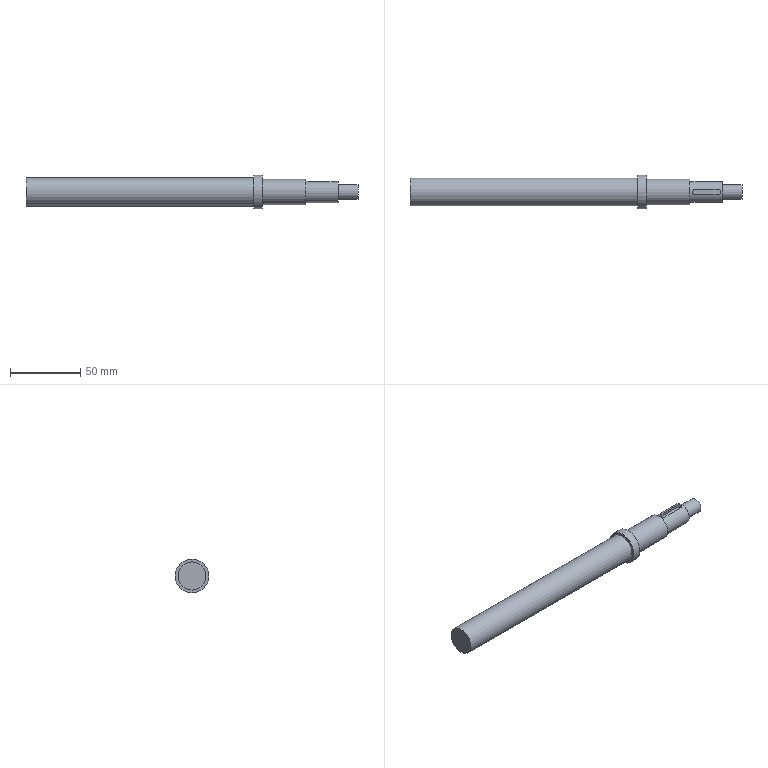Component | NX | LEAD_SCREW | 1 solid | 16 faces | volume 66645 mm3 | plane 9 | cylinder 7 | commonest cylinder face diameters 4 x2 15 x1 10.579 x1 18 x1 24 x1 20 x1